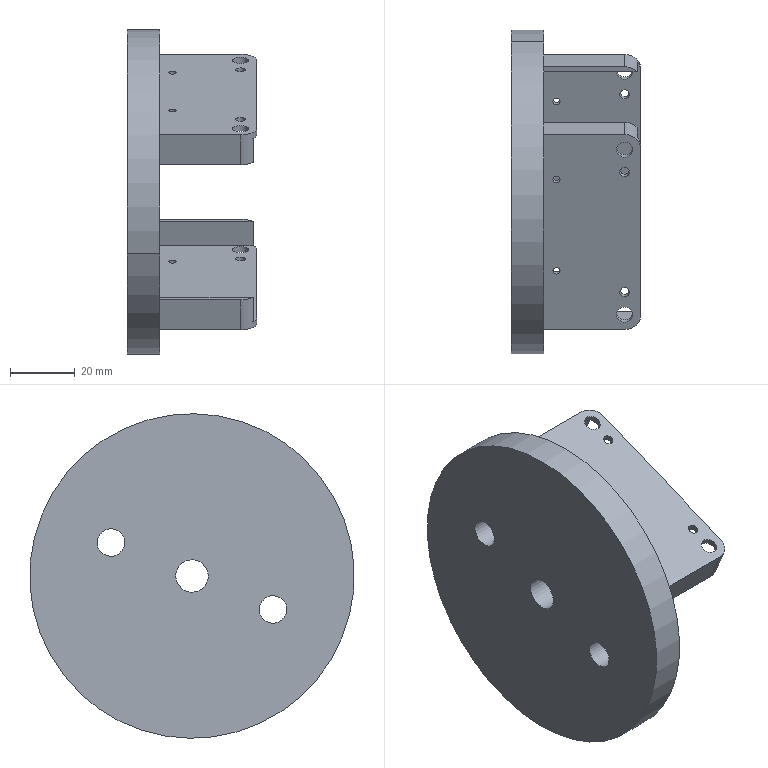Component | SolidWorks | Part1(1)-1 | 1 solid | 60 faces | volume 85538 mm3 | cylinder 36 | plane 20 | cone 4 | commonest cylinder face diameters 5 x8 2.2 x8 3 x8 10 x6 8.5 x4 100 x2